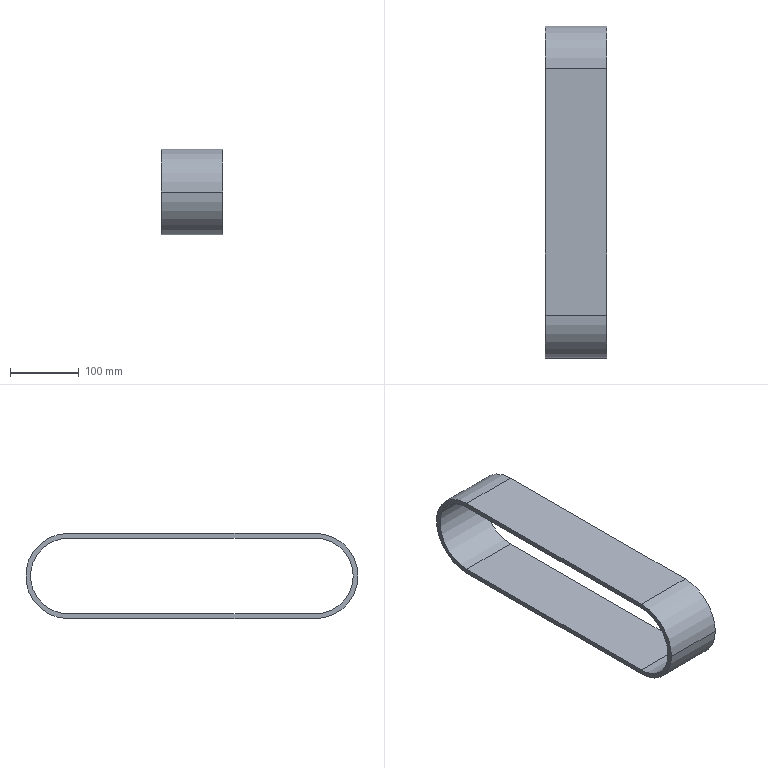Component | SolidWorks | LowerSideBeltXG-XG1-1_TractorBeltXG-XG1-1 | 1 solid | 12 faces | box 90 x 482.5 x 124 mm | volume 683277 mm3 | cylinder 6 | plane 6 | commonest cylinder face diameters 110 x3 124 x3
build123d program:
from build123d import *

# Parameters (mm, degrees)
EXTRUDE_THIN1_DEPTH = 45


with BuildPart() as part:
    # Sketch1 → Extrude-Thin1 (new, symmetric)
    with BuildSketch(Plane.XY):
        with BuildLine():
            Line((-358.5, 62), (0, 62))
            ThreePointArc((0, 62), (62, 0), (0, -62))
            Line((0, -62), (-358.5, -62))
            ThreePointArc((-358.5, -62), (-420.5, 0), (-358.5, 62))
        make_face()
        with BuildLine():
            Line((-358.5, 55), (0, 55))
            ThreePointArc((0, 55), (55, 0), (0, -55))
            Line((0, -55), (-358.5, -55))
            ThreePointArc((-358.5, -55), (-413.5, 0), (-358.5, 55))
        make_face(mode=Mode.SUBTRACT)
    extrude(amount=EXTRUDE_THIN1_DEPTH, both=True)


solid = part.part

# Placed as in the assembly
solid = solid.moved(Location((-246.22, 266.5, 114), (90, -90, 0)))
STEP:
#1=COLOUR_RGB('',0.7922,0.8196,0.9333);
#2=FILL_AREA_STYLE_COLOUR('',#1);
#3=FILL_AREA_STYLE('',(#2));
#4=SURFACE_STYLE_FILL_AREA(#3);
#5=SURFACE_SIDE_STYLE('',(#4));
#6=SURFACE_STYLE_USAGE(.BOTH.,#5);
#7=PRESENTATION_STYLE_ASSIGNMENT((#6));
#8=CARTESIAN_POINT('',(-7.922,10.492,6.654));
#9=VERTEX_POINT('',#8);
#10=CARTESIAN_POINT('',(-7.922,8.327,4.488));
#11=VERTEX_POINT('',#10);
#12=CARTESIAN_POINT('',(-7.922,10.492,4.488));
#13=DIRECTION('',(1.,0.,-0.));
#14=DIRECTION('',(0.,1.,0.));
#15=AXIS2_PLACEMENT_3D('',#12,#13,#14);
#16=CIRCLE('',#15,2.165);
#17=EDGE_CURVE('',#9,#11,#16,.T.);
#18=ORIENTED_EDGE('',*,*,#17,.T.);
#19=CARTESIAN_POINT('',(-11.465,8.327,4.488));
#20=VERTEX_POINT('',#19);
#21=CARTESIAN_POINT('',(-7.922,8.327,4.488));
#22=DIRECTION('',(-1.,-0.,0.));
#23=VECTOR('',#22,39.37);
#24=LINE('',#21,#23);
#25=EDGE_CURVE('',#11,#20,#24,.T.);
#26=ORIENTED_EDGE('',*,*,#25,.T.);
#27=CARTESIAN_POINT('',(-11.465,10.492,6.654));
#28=VERTEX_POINT('',#27);
#29=CARTESIAN_POINT('',(-11.465,10.492,4.488));
#30=DIRECTION('',(1.,0.,-0.));
#31=DIRECTION('',(0.,1.,0.));
#32=AXIS2_PLACEMENT_3D('',#29,#30,#31);
#33=CIRCLE('',#32,2.165);
#34=EDGE_CURVE('',#28,#20,#33,.T.);
#35=ORIENTED_EDGE('',*,*,#34,.F.);
#36=CARTESIAN_POINT('',(-7.922,10.492,6.654));
#37=DIRECTION('',(-1.,-0.,0.));
#38=VECTOR('',#37,39.37);
#39=LINE('',#36,#38);
#40=EDGE_CURVE('',#9,#28,#39,.T.);
#41=ORIENTED_EDGE('',*,*,#40,.F.);
#42=EDGE_LOOP('',(#18,#26,#35,#41));
#43=FACE_OUTER_BOUND('',#42,.T.);
#44=CARTESIAN_POINT('',(-7.922,10.492,4.488));
#45=DIRECTION('',(-1.,-0.,0.));
#46=DIRECTION('',(0.,-1.,-0.));
#47=AXIS2_PLACEMENT_3D('',#44,#45,#46);
#48=CYLINDRICAL_SURFACE('',#47,2.165);
#49=ADVANCED_FACE('',(#43),#48,.F.);
#50=CARTESIAN_POINT('',(-7.922,8.051,4.488));
#51=VERTEX_POINT('',#50);
#52=CARTESIAN_POINT('',(-7.922,10.492,2.047));
#53=VERTEX_POINT('',#52);
#54=CARTESIAN_POINT('',(-7.922,10.492,4.488));
#55=DIRECTION('',(1.,0.,-0.));
#56=DIRECTION('',(0.,1.,0.));
#57=AXIS2_PLACEMENT_3D('',#54,#55,#56);
#58=CIRCLE('',#57,2.441);
#59=EDGE_CURVE('',#51,#53,#58,.T.);
#60=ORIENTED_EDGE('',*,*,#59,.F.);
#61=CARTESIAN_POINT('',(-11.465,8.051,4.488));
#62=VERTEX_POINT('',#61);
#63=CARTESIAN_POINT('',(-7.922,8.051,4.488));
#64=DIRECTION('',(-1.,-0.,0.));
#65=VECTOR('',#64,39.37);
#66=LINE('',#63,#65);
#67=EDGE_CURVE('',#51,#62,#66,.T.);
#68=ORIENTED_EDGE('',*,*,#67,.T.);
#69=CARTESIAN_POINT('',(-11.465,10.492,2.047));
#70=VERTEX_POINT('',#69);
#71=CARTESIAN_POINT('',(-11.465,10.492,4.488));
#72=DIRECTION('',(1.,0.,-0.));
#73=DIRECTION('',(0.,1.,0.));
#74=AXIS2_PLACEMENT_3D('',#71,#72,#73);
#75=CIRCLE('',#74,2.441);
#76=EDGE_CURVE('',#62,#70,#75,.T.);
#77=ORIENTED_EDGE('',*,*,#76,.T.);
#78=CARTESIAN_POINT('',(-7.922,10.492,2.047));
#79=DIRECTION('',(-1.,-0.,0.));
#80=VECTOR('',#79,39.37);
#81=LINE('',#78,#80);
#82=EDGE_CURVE('',#53,#70,#81,.T.);
#83=ORIENTED_EDGE('',*,*,#82,.F.);
#84=EDGE_LOOP('',(#60,#68,#77,#83));
#85=FACE_OUTER_BOUND('',#84,.T.);
#86=CARTESIAN_POINT('',(-7.922,10.492,4.488));
#87=DIRECTION('',(-1.,-0.,0.));
#88=DIRECTION('',(0.,-1.,-0.));
#89=AXIS2_PLACEMENT_3D('',#86,#87,#88);
#90=CYLINDRICAL_SURFACE('',#89,2.441);
#91=ADVANCED_FACE('',(#85),#90,.T.);
#92=CARTESIAN_POINT('',(-7.922,24.606,2.047));
#93=VERTEX_POINT('',#92);
#94=CARTESIAN_POINT('',(-7.922,24.606,6.929));
#95=VERTEX_POINT('',#94);
#96=CARTESIAN_POINT('',(-7.922,24.606,4.488));
#97=DIRECTION('',(1.,0.,-0.));
#98=DIRECTION('',(0.,1.,0.));
#99=AXIS2_PLACEMENT_3D('',#96,#97,#98);
#100=CIRCLE('',#99,2.441);
#101=EDGE_CURVE('',#93,#95,#100,.T.);
#102=ORIENTED_EDGE('',*,*,#101,.T.);
#103=CARTESIAN_POINT('',(-7.922,10.492,6.929));
#104=VERTEX_POINT('',#103);
#105=CARTESIAN_POINT('',(-7.922,24.606,6.929));
#106=DIRECTION('',(0.,-1.,-0.));
#107=VECTOR('',#106,39.37);
#108=LINE('',#105,#107);
#109=EDGE_CURVE('',#95,#104,#108,.T.);
#110=ORIENTED_EDGE('',*,*,#109,.T.);
#111=CARTESIAN_POINT('',(-7.922,10.492,4.488));
#112=DIRECTION('',(1.,0.,-0.));
#113=DIRECTION('',(0.,1.,0.));
#114=AXIS2_PLACEMENT_3D('',#111,#112,#113);
#115=CIRCLE('',#114,2.441);
#116=EDGE_CURVE('',#104,#51,#115,.T.);
#117=ORIENTED_EDGE('',*,*,#116,.T.);
#118=ORIENTED_EDGE('',*,*,#59,.T.);
#119=CARTESIAN_POINT('',(-7.922,24.606,2.047));
#120=DIRECTION('',(-0.,1.,0.));
#121=VECTOR('',#120,39.37);
#122=LINE('',#119,#121);
#123=EDGE_CURVE('',#53,#93,#122,.T.);
#124=ORIENTED_EDGE('',*,*,#123,.T.);
#125=EDGE_LOOP('',(#102,#110,#117,#118,#124));
#126=FACE_OUTER_BOUND('',#125,.T.);
#127=CARTESIAN_POINT('',(-7.922,24.606,6.654));
#128=VERTEX_POINT('',#127);
#129=CARTESIAN_POINT('',(-7.922,24.606,6.654));
#130=DIRECTION('',(0.,-1.,-0.));
#131=VECTOR('',#130,39.37);
#132=LINE('',#129,#131);
#133=EDGE_CURVE('',#128,#9,#132,.T.);
#134=ORIENTED_EDGE('',*,*,#133,.F.);
#135=CARTESIAN_POINT('',(-7.922,24.606,2.323));
#136=VERTEX_POINT('',#135);
#137=CARTESIAN_POINT('',(-7.922,24.606,4.488));
#138=DIRECTION('',(1.,0.,-0.));
#139=DIRECTION('',(0.,1.,0.));
#140=AXIS2_PLACEMENT_3D('',#137,#138,#139);
#141=CIRCLE('',#140,2.165);
#142=EDGE_CURVE('',#136,#128,#141,.T.);
#143=ORIENTED_EDGE('',*,*,#142,.F.);
#144=CARTESIAN_POINT('',(-7.922,10.492,2.323));
#145=VERTEX_POINT('',#144);
#146=CARTESIAN_POINT('',(-7.922,24.606,2.323));
#147=DIRECTION('',(-0.,1.,0.));
#148=VECTOR('',#147,39.37);
#149=LINE('',#146,#148);
#150=EDGE_CURVE('',#145,#136,#149,.T.);
#151=ORIENTED_EDGE('',*,*,#150,.F.);
#152=CARTESIAN_POINT('',(-7.922,10.492,4.488));
#153=DIRECTION('',(1.,0.,-0.));
#154=DIRECTION('',(0.,1.,0.));
#155=AXIS2_PLACEMENT_3D('',#152,#153,#154);
#156=CIRCLE('',#155,2.165);
#157=EDGE_CURVE('',#11,#145,#156,.T.);
#158=ORIENTED_EDGE('',*,*,#157,.F.);
#159=ORIENTED_EDGE('',*,*,#17,.F.);
#160=EDGE_LOOP('',(#134,#143,#151,#158,#159));
#161=FACE_BOUND('',#160,.T.);
#162=CARTESIAN_POINT('',(-7.922,24.606,4.488));
#163=DIRECTION('',(1.,0.,-0.));
#164=DIRECTION('',(-0.,1.,0.));
#165=AXIS2_PLACEMENT_3D('',#162,#163,#164);
#166=PLANE('',#165);
#167=ADVANCED_FACE('',(#126,#161),#166,.T.);
#168=CARTESIAN_POINT('',(-11.465,24.606,2.047));
#169=VERTEX_POINT('',#168);
#170=CARTESIAN_POINT('',(-11.465,24.606,6.929));
#171=VERTEX_POINT('',#170);
#172=CARTESIAN_POINT('',(-11.465,24.606,4.488));
#173=DIRECTION('',(1.,0.,-0.));
#174=DIRECTION('',(0.,1.,0.));
#175=AXIS2_PLACEMENT_3D('',#172,#173,#174);
#176=CIRCLE('',#175,2.441);
#177=EDGE_CURVE('',#169,#171,#176,.T.);
#178=ORIENTED_EDGE('',*,*,#177,.F.);
#179=CARTESIAN_POINT('',(-11.465,24.606,2.047));
#180=DIRECTION('',(-0.,1.,0.));
#181=VECTOR('',#180,39.37);
#182=LINE('',#179,#181);
#183=EDGE_CURVE('',#70,#169,#182,.T.);
#184=ORIENTED_EDGE('',*,*,#183,.F.);
#185=ORIENTED_EDGE('',*,*,#76,.F.);
#186=CARTESIAN_POINT('',(-11.465,10.492,6.929));
#187=VERTEX_POINT('',#186);
#188=CARTESIAN_POINT('',(-11.465,10.492,4.488));
#189=DIRECTION('',(1.,0.,-0.));
#190=DIRECTION('',(0.,1.,0.));
#191=AXIS2_PLACEMENT_3D('',#188,#189,#190);
#192=CIRCLE('',#191,2.441);
#193=EDGE_CURVE('',#187,#62,#192,.T.);
#194=ORIENTED_EDGE('',*,*,#193,.F.);
#195=CARTESIAN_POINT('',(-11.465,24.606,6.929));
#196=DIRECTION('',(0.,-1.,-0.));
#197=VECTOR('',#196,39.37);
#198=LINE('',#195,#197);
#199=EDGE_CURVE('',#171,#187,#198,.T.);
#200=ORIENTED_EDGE('',*,*,#199,.F.);
#201=EDGE_LOOP('',(#178,#184,#185,#194,#200));
#202=FACE_OUTER_BOUND('',#201,.T.);
#203=CARTESIAN_POINT('',(-11.465,24.606,2.323));
#204=VERTEX_POINT('',#203);
#205=CARTESIAN_POINT('',(-11.465,24.606,6.654));
#206=VERTEX_POINT('',#205);
#207=CARTESIAN_POINT('',(-11.465,24.606,4.488));
#208=DIRECTION('',(1.,0.,-0.));
#209=DIRECTION('',(0.,1.,0.));
#210=AXIS2_PLACEMENT_3D('',#207,#208,#209);
#211=CIRCLE('',#210,2.165);
#212=EDGE_CURVE('',#204,#206,#211,.T.);
#213=ORIENTED_EDGE('',*,*,#212,.T.);
#214=CARTESIAN_POINT('',(-11.465,24.606,6.654));
#215=DIRECTION('',(0.,-1.,-0.));
#216=VECTOR('',#215,39.37);
#217=LINE('',#214,#216);
#218=EDGE_CURVE('',#206,#28,#217,.T.);
#219=ORIENTED_EDGE('',*,*,#218,.T.);
#220=ORIENTED_EDGE('',*,*,#34,.T.);
#221=CARTESIAN_POINT('',(-11.465,10.492,2.323));
#222=VERTEX_POINT('',#221);
#223=CARTESIAN_POINT('',(-11.465,10.492,4.488));
#224=DIRECTION('',(1.,0.,-0.));
#225=DIRECTION('',(0.,1.,0.));
#226=AXIS2_PLACEMENT_3D('',#223,#224,#225);
#227=CIRCLE('',#226,2.165);
#228=EDGE_CURVE('',#20,#222,#227,.T.);
#229=ORIENTED_EDGE('',*,*,#228,.T.);
#230=CARTESIAN_POINT('',(-11.465,24.606,2.323));
#231=DIRECTION('',(-0.,1.,0.));
#232=VECTOR('',#231,39.37);
#233=LINE('',#230,#232);
#234=EDGE_CURVE('',#222,#204,#233,.T.);
#235=ORIENTED_EDGE('',*,*,#234,.T.);
#236=EDGE_LOOP('',(#213,#219,#220,#229,#235));
#237=FACE_BOUND('',#236,.T.);
#238=CARTESIAN_POINT('',(-11.465,24.606,4.488));
#239=DIRECTION('',(1.,0.,-0.));
#240=DIRECTION('',(-0.,1.,0.));
#241=AXIS2_PLACEMENT_3D('',#238,#239,#240);
#242=PLANE('',#241);
#243=ADVANCED_FACE('',(#202,#237),#242,.F.);
#244=ORIENTED_EDGE('',*,*,#177,.T.);
#245=CARTESIAN_POINT('',(-7.922,24.606,6.929));
#246=DIRECTION('',(-1.,-0.,0.));
#247=VECTOR('',#246,39.37);
#248=LINE('',#245,#247);
#249=EDGE_CURVE('',#95,#171,#248,.T.);
#250=ORIENTED_EDGE('',*,*,#249,.F.);
#251=ORIENTED_EDGE('',*,*,#101,.F.);
#252=CARTESIAN_POINT('',(-7.922,24.606,2.047));
#253=DIRECTION('',(-1.,-0.,0.));
#254=VECTOR('',#253,39.37);
#255=LINE('',#252,#254);
#256=EDGE_CURVE('',#93,#169,#255,.T.);
#257=ORIENTED_EDGE('',*,*,#256,.T.);
#258=EDGE_LOOP('',(#244,#250,#251,#257));
#259=FACE_OUTER_BOUND('',#258,.T.);
#260=CARTESIAN_POINT('',(-7.922,24.606,4.488));
#261=DIRECTION('',(-1.,-0.,0.));
#262=DIRECTION('',(0.,-1.,-0.));
#263=AXIS2_PLACEMENT_3D('',#260,#261,#262);
#264=CYLINDRICAL_SURFACE('',#263,2.441);
#265=ADVANCED_FACE('',(#259),#264,.T.);
#266=ORIENTED_EDGE('',*,*,#199,.T.);
#267=CARTESIAN_POINT('',(-7.922,10.492,6.929));
#268=DIRECTION('',(-1.,-0.,0.));
#269=VECTOR('',#268,39.37);
#270=LINE('',#267,#269);
#271=EDGE_CURVE('',#104,#187,#270,.T.);
#272=ORIENTED_EDGE('',*,*,#271,.F.);
#273=ORIENTED_EDGE('',*,*,#109,.F.);
#274=ORIENTED_EDGE('',*,*,#249,.T.);
#275=EDGE_LOOP('',(#266,#272,#273,#274));
#276=FACE_OUTER_BOUND('',#275,.T.);
#277=CARTESIAN_POINT('',(-7.922,24.606,6.929));
#278=DIRECTION('',(-0.,0.,-1.));
#279=DIRECTION('',(-0.,1.,0.));
#280=AXIS2_PLACEMENT_3D('',#277,#278,#279);
#281=PLANE('',#280);
#282=ADVANCED_FACE('',(#276),#281,.F.);
#283=ORIENTED_EDGE('',*,*,#67,.F.);
#284=ORIENTED_EDGE('',*,*,#116,.F.);
#285=ORIENTED_EDGE('',*,*,#271,.T.);
#286=ORIENTED_EDGE('',*,*,#193,.T.);
#287=EDGE_LOOP('',(#283,#284,#285,#286));
#288=FACE_OUTER_BOUND('',#287,.T.);
#289=CARTESIAN_POINT('',(-7.922,10.492,4.488));
#290=DIRECTION('',(-1.,-0.,0.));
#291=DIRECTION('',(0.,-1.,-0.));
#292=AXIS2_PLACEMENT_3D('',#289,#290,#291);
#293=CYLINDRICAL_SURFACE('',#292,2.441);
#294=ADVANCED_FACE('',(#288),#293,.T.);
#295=ORIENTED_EDGE('',*,*,#183,.T.);
#296=ORIENTED_EDGE('',*,*,#256,.F.);
#297=ORIENTED_EDGE('',*,*,#123,.F.);
#298=ORIENTED_EDGE('',*,*,#82,.T.);
#299=EDGE_LOOP('',(#295,#296,#297,#298));
#300=FACE_OUTER_BOUND('',#299,.T.);
#301=CARTESIAN_POINT('',(-7.922,24.606,2.047));
#302=DIRECTION('',(0.,-0.,1.));
#303=DIRECTION('',(0.,-1.,-0.));
#304=AXIS2_PLACEMENT_3D('',#301,#302,#303);
#305=PLANE('',#304);
#306=ADVANCED_FACE('',(#300),#305,.F.);
#307=ORIENTED_EDGE('',*,*,#212,.F.);
#308=CARTESIAN_POINT('',(-7.922,24.606,2.323));
#309=DIRECTION('',(-1.,-0.,0.));
#310=VECTOR('',#309,39.37);
#311=LINE('',#308,#310);
#312=EDGE_CURVE('',#136,#204,#311,.T.);
#313=ORIENTED_EDGE('',*,*,#312,.F.);
#314=ORIENTED_EDGE('',*,*,#142,.T.);
#315=CARTESIAN_POINT('',(-7.922,24.606,6.654));
#316=DIRECTION('',(-1.,-0.,0.));
#317=VECTOR('',#316,39.37);
#318=LINE('',#315,#317);
#319=EDGE_CURVE('',#128,#206,#318,.T.);
#320=ORIENTED_EDGE('',*,*,#319,.T.);
#321=EDGE_LOOP('',(#307,#313,#314,#320));
#322=FACE_OUTER_BOUND('',#321,.T.);
#323=CARTESIAN_POINT('',(-7.922,24.606,4.488));
#324=DIRECTION('',(-1.,-0.,0.));
#325=DIRECTION('',(0.,-1.,-0.));
#326=AXIS2_PLACEMENT_3D('',#323,#324,#325);
#327=CYLINDRICAL_SURFACE('',#326,2.165);
#328=ADVANCED_FACE('',(#322),#327,.F.);
#329=ORIENTED_EDGE('',*,*,#218,.F.);
#330=ORIENTED_EDGE('',*,*,#319,.F.);
#331=ORIENTED_EDGE('',*,*,#133,.T.);
#332=ORIENTED_EDGE('',*,*,#40,.T.);
#333=EDGE_LOOP('',(#329,#330,#331,#332));
#334=FACE_OUTER_BOUND('',#333,.T.);
#335=CARTESIAN_POINT('',(-7.922,24.606,6.654));
#336=DIRECTION('',(-0.,0.,-1.));
#337=DIRECTION('',(-0.,1.,0.));
#338=AXIS2_PLACEMENT_3D('',#335,#336,#337);
#339=PLANE('',#338);
#340=ADVANCED_FACE('',(#334),#339,.T.);
#341=ORIENTED_EDGE('',*,*,#25,.F.);
#342=ORIENTED_EDGE('',*,*,#157,.T.);
#343=CARTESIAN_POINT('',(-7.922,10.492,2.323));
#344=DIRECTION('',(-1.,-0.,0.));
#345=VECTOR('',#344,39.37);
#346=LINE('',#343,#345);
#347=EDGE_CURVE('',#145,#222,#346,.T.);
#348=ORIENTED_EDGE('',*,*,#347,.T.);
#349=ORIENTED_EDGE('',*,*,#228,.F.);
#350=EDGE_LOOP('',(#341,#342,#348,#349));
#351=FACE_OUTER_BOUND('',#350,.T.);
#352=CARTESIAN_POINT('',(-7.922,10.492,4.488));
#353=DIRECTION('',(-1.,-0.,0.));
#354=DIRECTION('',(0.,-1.,-0.));
#355=AXIS2_PLACEMENT_3D('',#352,#353,#354);
#356=CYLINDRICAL_SURFACE('',#355,2.165);
#357=ADVANCED_FACE('',(#351),#356,.F.);
#358=ORIENTED_EDGE('',*,*,#234,.F.);
#359=ORIENTED_EDGE('',*,*,#347,.F.);
#360=ORIENTED_EDGE('',*,*,#150,.T.);
#361=ORIENTED_EDGE('',*,*,#312,.T.);
#362=EDGE_LOOP('',(#358,#359,#360,#361));
#363=FACE_OUTER_BOUND('',#362,.T.);
#364=CARTESIAN_POINT('',(-7.922,24.606,2.323));
#365=DIRECTION('',(0.,-0.,1.));
#366=DIRECTION('',(0.,-1.,-0.));
#367=AXIS2_PLACEMENT_3D('',#364,#365,#366);
#368=PLANE('',#367);
#369=ADVANCED_FACE('',(#363),#368,.T.);
#370=CLOSED_SHELL('',(#49,#91,#167,#243,#265,#282,#294,#306,#328,#340,#357,#369));
#371=MANIFOLD_SOLID_BREP('',#370);
#372=STYLED_ITEM('',(#7),#371);
#373=PRESENTATION_LAYER_ASSIGNMENT('','',(#372));
#374=(LENGTH_UNIT()NAMED_UNIT(*)SI_UNIT($,.METRE.));
#375=LENGTH_MEASURE_WITH_UNIT(LENGTH_MEASURE(0.0254),#374);
#376=DIMENSIONAL_EXPONENTS(1.,0.,0.,0.,0.,0.,0.);
#377=(CONVERSION_BASED_UNIT('',#375)LENGTH_UNIT()NAMED_UNIT(#376));
#378=UNCERTAINTY_MEASURE_WITH_UNIT(LENGTH_MEASURE(0.00001),#377,'','');
#379=(NAMED_UNIT(*)PLANE_ANGLE_UNIT()SI_UNIT($,.RADIAN.));
#380=(NAMED_UNIT(*)SI_UNIT($,.STERADIAN.)SOLID_ANGLE_UNIT());
#381=(GEOMETRIC_REPRESENTATION_CONTEXT(3)GLOBAL_UNCERTAINTY_ASSIGNED_CONTEXT((#378))GLOBAL_UNIT_ASSIGNED_CONTEXT((#377,#379,#380))REPRESENTATION_CONTEXT('',''));
#382=MECHANICAL_DESIGN_GEOMETRIC_PRESENTATION_REPRESENTATION('',(#372),#381);
#383=CARTESIAN_POINT('',(0.,0.,0.));
#384=DIRECTION('',(0.,0.,1.));
#385=DIRECTION('',(1.,0.,0.));
#386=AXIS2_PLACEMENT_3D('',#383,#384,#385);
#387=(LENGTH_UNIT()NAMED_UNIT(*)SI_UNIT($,.METRE.));
#388=LENGTH_MEASURE_WITH_UNIT(LENGTH_MEASURE(0.0254),#387);
#389=DIMENSIONAL_EXPONENTS(1.,0.,0.,0.,0.,0.,0.);
#390=(CONVERSION_BASED_UNIT('',#388)LENGTH_UNIT()NAMED_UNIT(#389));
#391=UNCERTAINTY_MEASURE_WITH_UNIT(LENGTH_MEASURE(0.00001),#390,'','');
#392=(NAMED_UNIT(*)PLANE_ANGLE_UNIT()SI_UNIT($,.RADIAN.));
#393=(NAMED_UNIT(*)SI_UNIT($,.STERADIAN.)SOLID_ANGLE_UNIT());
#394=(GEOMETRIC_REPRESENTATION_CONTEXT(3)GLOBAL_UNCERTAINTY_ASSIGNED_CONTEXT((#391))GLOBAL_UNIT_ASSIGNED_CONTEXT((#390,#392,#393))REPRESENTATION_CONTEXT('',''));
#395=ADVANCED_BREP_SHAPE_REPRESENTATION('',(#371,#386),#394);